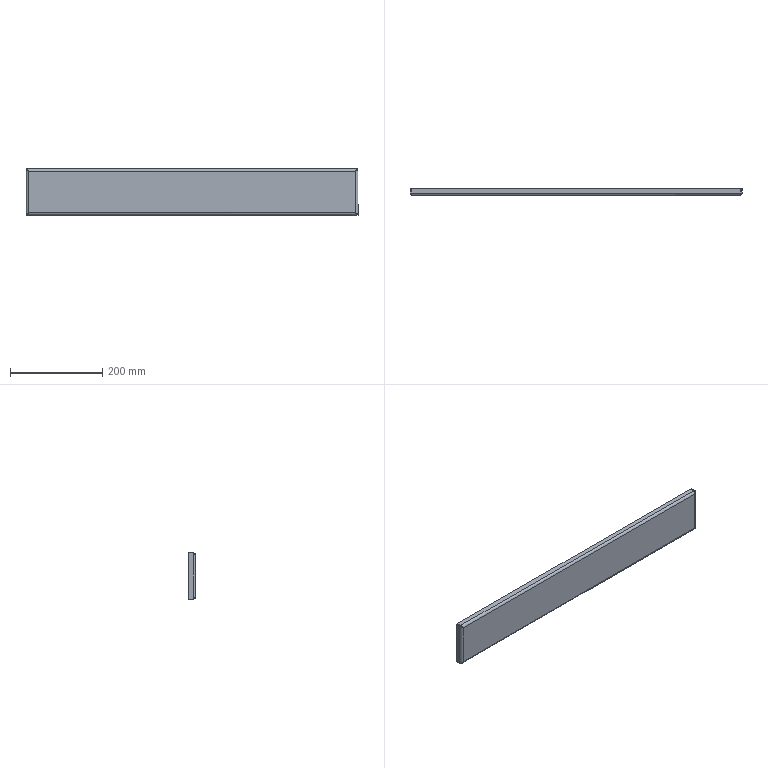Component | SolidWorks | BoxWelding-1_BottomSupport-2 | 1 solid | 38 faces | volume 267144 mm3 | plane 22 | spline 8 | cylinder 8 | commonest cylinder face diameters 10 x4 4 x4